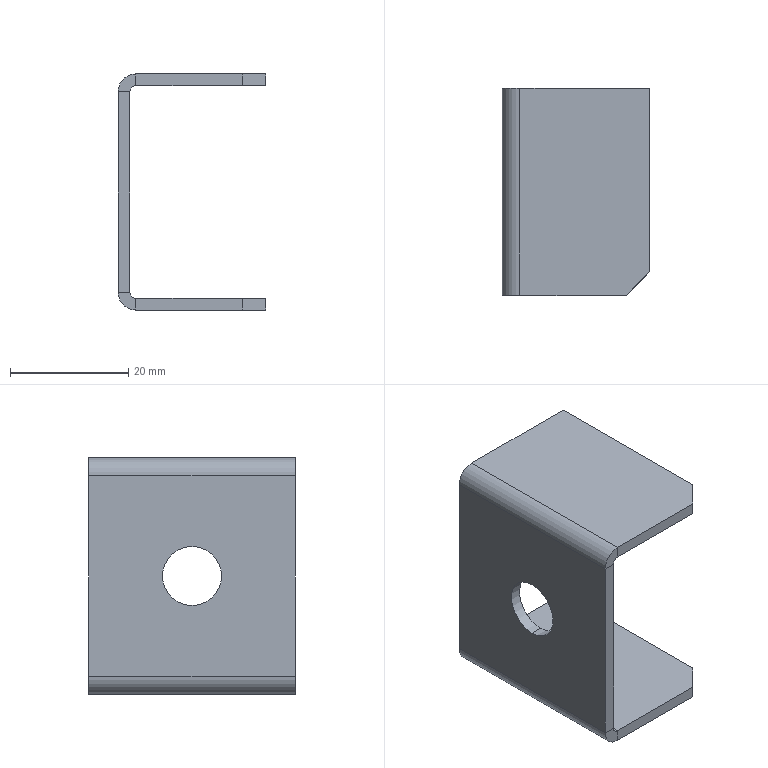Component | SolidWorks | GroundingDeviceAssembly-1_GroundingDevice-1 | 1 solid | 26 faces | box 25 x 35 x 40 mm | volume 5711 mm3 | plane 20 | cylinder 6 | commonest cylinder face diameters 10 x2 6 x2 2 x2
STEP:
#1=CARTESIAN_POINT('',(29.337,-7.169,9.724));
#2=VERTEX_POINT('',#1);
#3=CARTESIAN_POINT('',(29.337,-7.169,9.331));
#4=VERTEX_POINT('',#3);
#5=CARTESIAN_POINT('',(29.337,-7.169,9.528));
#6=DIRECTION('',(1.,0.,-0.));
#7=DIRECTION('',(0.,0.,-1.));
#8=AXIS2_PLACEMENT_3D('',#5,#6,#7);
#9=CIRCLE('',#8,0.1969);
#10=EDGE_CURVE('',#2,#4,#9,.T.);
#11=ORIENTED_EDGE('',*,*,#10,.T.);
#12=CARTESIAN_POINT('',(29.258,-7.169,9.331));
#13=VERTEX_POINT('',#12);
#14=CARTESIAN_POINT('',(29.376,-7.169,9.331));
#15=DIRECTION('',(-1.,-0.,0.));
#16=VECTOR('',#15,39.37);
#17=LINE('',#14,#16);
#18=EDGE_CURVE('',#4,#13,#17,.T.);
#19=ORIENTED_EDGE('',*,*,#18,.T.);
#20=CARTESIAN_POINT('',(29.258,-7.169,9.724));
#21=VERTEX_POINT('',#20);
#22=CARTESIAN_POINT('',(29.258,-7.169,9.528));
#23=DIRECTION('',(-1.,-0.,0.));
#24=DIRECTION('',(0.,0.,1.));
#25=AXIS2_PLACEMENT_3D('',#22,#23,#24);
#26=CIRCLE('',#25,0.1969);
#27=EDGE_CURVE('',#13,#21,#26,.T.);
#28=ORIENTED_EDGE('',*,*,#27,.T.);
#29=CARTESIAN_POINT('',(29.376,-7.169,9.724));
#30=DIRECTION('',(-1.,-0.,0.));
#31=VECTOR('',#30,39.37);
#32=LINE('',#29,#31);
#33=EDGE_CURVE('',#2,#21,#32,.T.);
#34=ORIENTED_EDGE('',*,*,#33,.F.);
#35=EDGE_LOOP('',(#11,#19,#28,#34));
#36=FACE_OUTER_BOUND('',#35,.T.);
#37=CARTESIAN_POINT('',(29.376,-7.169,9.528));
#38=DIRECTION('',(-1.,-0.,0.));
#39=DIRECTION('',(0.,0.,1.));
#40=AXIS2_PLACEMENT_3D('',#37,#38,#39);
#41=CYLINDRICAL_SURFACE('',#40,0.1969);
#42=ADVANCED_FACE('',(#36),#41,.F.);
#43=CARTESIAN_POINT('',(29.258,-7.169,9.528));
#44=DIRECTION('',(-1.,-0.,0.));
#45=DIRECTION('',(0.,0.,1.));
#46=AXIS2_PLACEMENT_3D('',#43,#44,#45);
#47=CIRCLE('',#46,0.1969);
#48=EDGE_CURVE('',#21,#13,#47,.T.);
#49=ORIENTED_EDGE('',*,*,#48,.F.);
#50=ORIENTED_EDGE('',*,*,#27,.F.);
#51=EDGE_LOOP('',(#49,#50));
#52=FACE_BOUND('',#51,.T.);
#53=CARTESIAN_POINT('',(29.258,-6.481,8.858));
#54=VERTEX_POINT('',#53);
#55=CARTESIAN_POINT('',(29.258,-7.858,8.858));
#56=VERTEX_POINT('',#55);
#57=CARTESIAN_POINT('',(29.258,-6.481,8.858));
#58=DIRECTION('',(0.,-1.,0.));
#59=VECTOR('',#58,39.37);
#60=LINE('',#57,#59);
#61=EDGE_CURVE('',#54,#56,#60,.T.);
#62=ORIENTED_EDGE('',*,*,#61,.T.);
#63=CARTESIAN_POINT('',(29.258,-7.858,10.197));
#64=VERTEX_POINT('',#63);
#65=CARTESIAN_POINT('',(29.258,-7.858,10.315));
#66=DIRECTION('',(-0.,-0.,-1.));
#67=VECTOR('',#66,39.37);
#68=LINE('',#65,#67);
#69=EDGE_CURVE('',#64,#56,#68,.T.);
#70=ORIENTED_EDGE('',*,*,#69,.F.);
#71=CARTESIAN_POINT('',(29.258,-6.481,10.197));
#72=VERTEX_POINT('',#71);
#73=CARTESIAN_POINT('',(29.258,-7.858,10.197));
#74=DIRECTION('',(-0.,1.,-0.));
#75=VECTOR('',#74,39.37);
#76=LINE('',#73,#75);
#77=EDGE_CURVE('',#64,#72,#76,.T.);
#78=ORIENTED_EDGE('',*,*,#77,.T.);
#79=CARTESIAN_POINT('',(29.258,-6.481,10.315));
#80=DIRECTION('',(0.,0.,1.));
#81=VECTOR('',#80,39.37);
#82=LINE('',#79,#81);
#83=EDGE_CURVE('',#54,#72,#82,.T.);
#84=ORIENTED_EDGE('',*,*,#83,.F.);
#85=EDGE_LOOP('',(#62,#70,#78,#84));
#86=FACE_OUTER_BOUND('',#85,.T.);
#87=CARTESIAN_POINT('',(29.258,-7.858,8.74));
#88=DIRECTION('',(1.,0.,-0.));
#89=DIRECTION('',(-0.,-0.,-1.));
#90=AXIS2_PLACEMENT_3D('',#87,#88,#89);
#91=PLANE('',#90);
#92=ADVANCED_FACE('',(#52,#86),#91,.F.);
#93=ORIENTED_EDGE('',*,*,#10,.F.);
#94=CARTESIAN_POINT('',(29.337,-7.169,9.528));
#95=DIRECTION('',(1.,0.,-0.));
#96=DIRECTION('',(0.,0.,-1.));
#97=AXIS2_PLACEMENT_3D('',#94,#95,#96);
#98=CIRCLE('',#97,0.1969);
#99=EDGE_CURVE('',#4,#2,#98,.T.);
#100=ORIENTED_EDGE('',*,*,#99,.F.);
#101=EDGE_LOOP('',(#93,#100));
#102=FACE_BOUND('',#101,.T.);
#103=CARTESIAN_POINT('',(29.337,-7.858,10.197));
#104=VERTEX_POINT('',#103);
#105=CARTESIAN_POINT('',(29.337,-7.858,8.858));
#106=VERTEX_POINT('',#105);
#107=CARTESIAN_POINT('',(29.337,-7.858,10.315));
#108=DIRECTION('',(-0.,-0.,-1.));
#109=VECTOR('',#108,39.37);
#110=LINE('',#107,#109);
#111=EDGE_CURVE('',#104,#106,#110,.T.);
#112=ORIENTED_EDGE('',*,*,#111,.T.);
#113=CARTESIAN_POINT('',(29.337,-6.481,8.858));
#114=VERTEX_POINT('',#113);
#115=CARTESIAN_POINT('',(29.337,-6.481,8.858));
#116=DIRECTION('',(0.,-1.,0.));
#117=VECTOR('',#116,39.37);
#118=LINE('',#115,#117);
#119=EDGE_CURVE('',#114,#106,#118,.T.);
#120=ORIENTED_EDGE('',*,*,#119,.F.);
#121=CARTESIAN_POINT('',(29.337,-6.481,10.197));
#122=VERTEX_POINT('',#121);
#123=CARTESIAN_POINT('',(29.337,-6.481,10.315));
#124=DIRECTION('',(0.,0.,1.));
#125=VECTOR('',#124,39.37);
#126=LINE('',#123,#125);
#127=EDGE_CURVE('',#114,#122,#126,.T.);
#128=ORIENTED_EDGE('',*,*,#127,.T.);
#129=CARTESIAN_POINT('',(29.337,-7.858,10.197));
#130=DIRECTION('',(-0.,1.,-0.));
#131=VECTOR('',#130,39.37);
#132=LINE('',#129,#131);
#133=EDGE_CURVE('',#104,#122,#132,.T.);
#134=ORIENTED_EDGE('',*,*,#133,.F.);
#135=EDGE_LOOP('',(#112,#120,#128,#134));
#136=FACE_OUTER_BOUND('',#135,.T.);
#137=CARTESIAN_POINT('',(29.337,-7.858,8.74));
#138=DIRECTION('',(1.,0.,-0.));
#139=DIRECTION('',(-0.,-0.,-1.));
#140=AXIS2_PLACEMENT_3D('',#137,#138,#139);
#141=PLANE('',#140);
#142=ADVANCED_FACE('',(#102,#136),#141,.T.);
#143=ORIENTED_EDGE('',*,*,#127,.F.);
#144=CARTESIAN_POINT('',(29.337,-6.481,8.858));
#145=DIRECTION('',(-1.,-0.,0.));
#146=VECTOR('',#145,39.37);
#147=LINE('',#144,#146);
#148=EDGE_CURVE('',#114,#54,#147,.T.);
#149=ORIENTED_EDGE('',*,*,#148,.T.);
#150=ORIENTED_EDGE('',*,*,#83,.T.);
#151=CARTESIAN_POINT('',(29.337,-6.481,10.197));
#152=DIRECTION('',(-1.,-0.,-0.));
#153=VECTOR('',#152,39.37);
#154=LINE('',#151,#153);
#155=EDGE_CURVE('',#122,#72,#154,.T.);
#156=ORIENTED_EDGE('',*,*,#155,.F.);
#157=EDGE_LOOP('',(#143,#149,#150,#156));
#158=FACE_OUTER_BOUND('',#157,.T.);
#159=CARTESIAN_POINT('',(29.258,-6.481,10.315));
#160=DIRECTION('',(-0.,1.,-0.));
#161=DIRECTION('',(1.,0.,-0.));
#162=AXIS2_PLACEMENT_3D('',#159,#160,#161);
#163=PLANE('',#162);
#164=ADVANCED_FACE('',(#158),#163,.T.);
#165=CARTESIAN_POINT('',(29.337,-7.858,8.858));
#166=DIRECTION('',(-1.,-0.,0.));
#167=VECTOR('',#166,39.37);
#168=LINE('',#165,#167);
#169=EDGE_CURVE('',#106,#56,#168,.T.);
#170=ORIENTED_EDGE('',*,*,#169,.F.);
#171=ORIENTED_EDGE('',*,*,#111,.F.);
#172=CARTESIAN_POINT('',(29.337,-7.858,10.197));
#173=DIRECTION('',(-1.,-0.,-0.));
#174=VECTOR('',#173,39.37);
#175=LINE('',#172,#174);
#176=EDGE_CURVE('',#104,#64,#175,.T.);
#177=ORIENTED_EDGE('',*,*,#176,.T.);
#178=ORIENTED_EDGE('',*,*,#69,.T.);
#179=EDGE_LOOP('',(#170,#171,#177,#178));
#180=FACE_OUTER_BOUND('',#179,.T.);
#181=CARTESIAN_POINT('',(29.258,-7.858,10.315));
#182=DIRECTION('',(0.,-1.,0.));
#183=DIRECTION('',(-1.,-0.,0.));
#184=AXIS2_PLACEMENT_3D('',#181,#182,#183);
#185=PLANE('',#184);
#186=ADVANCED_FACE('',(#180),#185,.T.);
#187=CARTESIAN_POINT('',(29.376,-6.481,10.236));
#188=VERTEX_POINT('',#187);
#189=CARTESIAN_POINT('',(29.376,-6.481,10.315));
#190=VERTEX_POINT('',#189);
#191=CARTESIAN_POINT('',(29.376,-6.481,10.315));
#192=DIRECTION('',(-0.,-0.,1.));
#193=VECTOR('',#192,39.37);
#194=LINE('',#191,#193);
#195=EDGE_CURVE('',#188,#190,#194,.T.);
#196=ORIENTED_EDGE('',*,*,#195,.F.);
#197=CARTESIAN_POINT('',(29.376,-6.481,10.197));
#198=DIRECTION('',(-0.,1.,-0.));
#199=DIRECTION('',(-1.,0.,0.));
#200=AXIS2_PLACEMENT_3D('',#197,#198,#199);
#201=CIRCLE('',#200,0.03937);
#202=EDGE_CURVE('',#122,#188,#201,.T.);
#203=ORIENTED_EDGE('',*,*,#202,.F.);
#204=ORIENTED_EDGE('',*,*,#155,.T.);
#205=CARTESIAN_POINT('',(29.376,-6.481,10.197));
#206=DIRECTION('',(-0.,1.,-0.));
#207=DIRECTION('',(-1.,0.,0.));
#208=AXIS2_PLACEMENT_3D('',#205,#206,#207);
#209=CIRCLE('',#208,0.1181);
#210=EDGE_CURVE('',#72,#190,#209,.T.);
#211=ORIENTED_EDGE('',*,*,#210,.T.);
#212=EDGE_LOOP('',(#196,#203,#204,#211));
#213=FACE_OUTER_BOUND('',#212,.T.);
#214=CARTESIAN_POINT('',(29.376,-6.481,10.197));
#215=DIRECTION('',(-0.,1.,-0.));
#216=DIRECTION('',(1.,0.,-0.));
#217=AXIS2_PLACEMENT_3D('',#214,#215,#216);
#218=PLANE('',#217);
#219=ADVANCED_FACE('',(#213),#218,.T.);
#220=CARTESIAN_POINT('',(29.376,-7.858,10.236));
#221=VERTEX_POINT('',#220);
#222=CARTESIAN_POINT('',(29.376,-7.858,10.197));
#223=DIRECTION('',(0.,-1.,0.));
#224=DIRECTION('',(-1.,0.,0.));
#225=AXIS2_PLACEMENT_3D('',#222,#223,#224);
#226=CIRCLE('',#225,0.03937);
#227=EDGE_CURVE('',#221,#104,#226,.T.);
#228=ORIENTED_EDGE('',*,*,#227,.F.);
#229=CARTESIAN_POINT('',(29.376,-7.858,10.315));
#230=VERTEX_POINT('',#229);
#231=CARTESIAN_POINT('',(29.376,-7.858,10.236));
#232=DIRECTION('',(-0.,-0.,1.));
#233=VECTOR('',#232,39.37);
#234=LINE('',#231,#233);
#235=EDGE_CURVE('',#221,#230,#234,.T.);
#236=ORIENTED_EDGE('',*,*,#235,.T.);
#237=CARTESIAN_POINT('',(29.376,-7.858,10.197));
#238=DIRECTION('',(0.,-1.,0.));
#239=DIRECTION('',(-1.,0.,0.));
#240=AXIS2_PLACEMENT_3D('',#237,#238,#239);
#241=CIRCLE('',#240,0.1181);
#242=EDGE_CURVE('',#230,#64,#241,.T.);
#243=ORIENTED_EDGE('',*,*,#242,.T.);
#244=ORIENTED_EDGE('',*,*,#176,.F.);
#245=EDGE_LOOP('',(#228,#236,#243,#244));
#246=FACE_OUTER_BOUND('',#245,.T.);
#247=CARTESIAN_POINT('',(29.376,-7.858,10.197));
#248=DIRECTION('',(-0.,1.,-0.));
#249=DIRECTION('',(1.,0.,-0.));
#250=AXIS2_PLACEMENT_3D('',#247,#248,#249);
#251=PLANE('',#250);
#252=ADVANCED_FACE('',(#246),#251,.F.);
#253=ORIENTED_EDGE('',*,*,#77,.F.);
#254=ORIENTED_EDGE('',*,*,#242,.F.);
#255=CARTESIAN_POINT('',(29.376,-6.481,10.315));
#256=DIRECTION('',(-0.,1.,-0.));
#257=VECTOR('',#256,39.37);
#258=LINE('',#255,#257);
#259=EDGE_CURVE('',#230,#190,#258,.T.);
#260=ORIENTED_EDGE('',*,*,#259,.T.);
#261=ORIENTED_EDGE('',*,*,#210,.F.);
#262=EDGE_LOOP('',(#253,#254,#260,#261));
#263=FACE_OUTER_BOUND('',#262,.T.);
#264=CARTESIAN_POINT('',(29.376,-7.858,10.197));
#265=DIRECTION('',(0.,-1.,0.));
#266=DIRECTION('',(0.,0.,1.));
#267=AXIS2_PLACEMENT_3D('',#264,#265,#266);
#268=CYLINDRICAL_SURFACE('',#267,0.1181);
#269=ADVANCED_FACE('',(#263),#268,.T.);
#270=ORIENTED_EDGE('',*,*,#133,.T.);
#271=ORIENTED_EDGE('',*,*,#202,.T.);
#272=CARTESIAN_POINT('',(29.376,-6.481,10.236));
#273=DIRECTION('',(0.,-1.,0.));
#274=VECTOR('',#273,39.37);
#275=LINE('',#272,#274);
#276=EDGE_CURVE('',#188,#221,#275,.T.);
#277=ORIENTED_EDGE('',*,*,#276,.T.);
#278=ORIENTED_EDGE('',*,*,#227,.T.);
#279=EDGE_LOOP('',(#270,#271,#277,#278));
#280=FACE_OUTER_BOUND('',#279,.T.);
#281=CARTESIAN_POINT('',(29.376,-7.858,10.197));
#282=DIRECTION('',(0.,-1.,0.));
#283=DIRECTION('',(0.,0.,1.));
#284=AXIS2_PLACEMENT_3D('',#281,#282,#283);
#285=CYLINDRICAL_SURFACE('',#284,0.03937);
#286=ADVANCED_FACE('',(#280),#285,.F.);
#287=ORIENTED_EDGE('',*,*,#195,.T.);
#288=CARTESIAN_POINT('',(30.242,-6.481,10.315));
#289=VERTEX_POINT('',#288);
#290=CARTESIAN_POINT('',(30.242,-6.481,10.315));
#291=DIRECTION('',(-1.,-0.,-0.));
#292=VECTOR('',#291,39.37);
#293=LINE('',#290,#292);
#294=EDGE_CURVE('',#289,#190,#293,.T.);
#295=ORIENTED_EDGE('',*,*,#294,.F.);
#296=CARTESIAN_POINT('',(30.242,-6.481,10.236));
#297=VERTEX_POINT('',#296);
#298=CARTESIAN_POINT('',(30.242,-6.481,10.315));
#299=DIRECTION('',(0.,0.,-1.));
#300=VECTOR('',#299,39.37);
#301=LINE('',#298,#300);
#302=EDGE_CURVE('',#289,#297,#301,.T.);
#303=ORIENTED_EDGE('',*,*,#302,.T.);
#304=CARTESIAN_POINT('',(29.337,-6.481,10.236));
#305=DIRECTION('',(-1.,-0.,-0.));
#306=VECTOR('',#305,39.37);
#307=LINE('',#304,#306);
#308=EDGE_CURVE('',#297,#188,#307,.T.);
#309=ORIENTED_EDGE('',*,*,#308,.T.);
#310=EDGE_LOOP('',(#287,#295,#303,#309));
#311=FACE_OUTER_BOUND('',#310,.T.);
#312=CARTESIAN_POINT('',(29.337,-6.481,10.315));
#313=DIRECTION('',(0.,-1.,-0.));
#314=DIRECTION('',(-0.,0.,-1.));
#315=AXIS2_PLACEMENT_3D('',#312,#313,#314);
#316=PLANE('',#315);
#317=ADVANCED_FACE('',(#311),#316,.F.);
#318=CARTESIAN_POINT('',(30.085,-7.858,10.236));
#319=VERTEX_POINT('',#318);
#320=CARTESIAN_POINT('',(30.242,-7.858,10.236));
#321=DIRECTION('',(1.,0.,0.));
#322=VECTOR('',#321,39.37);
#323=LINE('',#320,#322);
#324=EDGE_CURVE('',#221,#319,#323,.T.);
#325=ORIENTED_EDGE('',*,*,#324,.T.);
#326=CARTESIAN_POINT('',(30.085,-7.858,10.315));
#327=VERTEX_POINT('',#326);
#328=CARTESIAN_POINT('',(30.085,-7.858,10.315));
#329=DIRECTION('',(-0.,-0.,1.));
#330=VECTOR('',#329,39.37);
#331=LINE('',#328,#330);
#332=EDGE_CURVE('',#319,#327,#331,.T.);
#333=ORIENTED_EDGE('',*,*,#332,.T.);
#334=CARTESIAN_POINT('',(30.242,-7.858,10.315));
#335=DIRECTION('',(1.,0.,0.));
#336=VECTOR('',#335,39.37);
#337=LINE('',#334,#336);
#338=EDGE_CURVE('',#230,#327,#337,.T.);
#339=ORIENTED_EDGE('',*,*,#338,.F.);
#340=ORIENTED_EDGE('',*,*,#235,.F.);
#341=EDGE_LOOP('',(#325,#333,#339,#340));
#342=FACE_OUTER_BOUND('',#341,.T.);
#343=CARTESIAN_POINT('',(30.242,-7.858,10.315));
#344=DIRECTION('',(-0.,1.,0.));
#345=DIRECTION('',(0.,-0.,1.));
#346=AXIS2_PLACEMENT_3D('',#343,#344,#345);
#347=PLANE('',#346);
#348=ADVANCED_FACE('',(#342),#347,.F.);
#349=ORIENTED_EDGE('',*,*,#338,.T.);
#350=CARTESIAN_POINT('',(30.242,-7.701,10.315));
#351=VERTEX_POINT('',#350);
#352=CARTESIAN_POINT('',(30.242,-7.701,10.315));
#353=DIRECTION('',(0.7071,0.7071,0.));
#354=VECTOR('',#353,39.37);
#355=LINE('',#352,#354);
#356=EDGE_CURVE('',#327,#351,#355,.T.);
#357=ORIENTED_EDGE('',*,*,#356,.T.);
#358=CARTESIAN_POINT('',(30.242,-6.481,10.315));
#359=DIRECTION('',(-0.,1.,-0.));
#360=VECTOR('',#359,39.37);
#361=LINE('',#358,#360);
#362=EDGE_CURVE('',#351,#289,#361,.T.);
#363=ORIENTED_EDGE('',*,*,#362,.T.);
#364=ORIENTED_EDGE('',*,*,#294,.T.);
#365=ORIENTED_EDGE('',*,*,#259,.F.);
#366=EDGE_LOOP('',(#349,#357,#363,#364,#365));
#367=FACE_OUTER_BOUND('',#366,.T.);
#368=CARTESIAN_POINT('',(30.242,-6.481,10.315));
#369=DIRECTION('',(0.,0.,-1.));
#370=DIRECTION('',(-1.,-0.,-0.));
#371=AXIS2_PLACEMENT_3D('',#368,#369,#370);
#372=PLANE('',#371);
#373=ADVANCED_FACE('',(#367),#372,.F.);
#374=CARTESIAN_POINT('',(30.242,-7.701,10.236));
#375=VERTEX_POINT('',#374);
#376=CARTESIAN_POINT('',(30.242,-6.481,10.236));
#377=DIRECTION('',(-0.,1.,-0.));
#378=VECTOR('',#377,39.37);
#379=LINE('',#376,#378);
#380=EDGE_CURVE('',#375,#297,#379,.T.);
#381=ORIENTED_EDGE('',*,*,#380,.F.);
#382=CARTESIAN_POINT('',(30.852,-7.091,10.236));
#383=DIRECTION('',(-0.7071,-0.7071,-0.));
#384=VECTOR('',#383,39.37);
#385=LINE('',#382,#384);
#386=EDGE_CURVE('',#375,#319,#385,.T.);
#387=ORIENTED_EDGE('',*,*,#386,.T.);
#388=ORIENTED_EDGE('',*,*,#324,.F.);
#389=ORIENTED_EDGE('',*,*,#276,.F.);
#390=ORIENTED_EDGE('',*,*,#308,.F.);
#391=EDGE_LOOP('',(#381,#387,#388,#389,#390));
#392=FACE_OUTER_BOUND('',#391,.T.);
#393=CARTESIAN_POINT('',(30.242,-6.481,10.236));
#394=DIRECTION('',(0.,0.,-1.));
#395=DIRECTION('',(-1.,-0.,-0.));
#396=AXIS2_PLACEMENT_3D('',#393,#394,#395);
#397=PLANE('',#396);
#398=ADVANCED_FACE('',(#392),#397,.T.);
#399=ORIENTED_EDGE('',*,*,#362,.F.);
#400=CARTESIAN_POINT('',(30.242,-7.701,10.315));
#401=DIRECTION('',(0.,0.,-1.));
#402=VECTOR('',#401,39.37);
#403=LINE('',#400,#402);
#404=EDGE_CURVE('',#351,#375,#403,.T.);
#405=ORIENTED_EDGE('',*,*,#404,.T.);
#406=ORIENTED_EDGE('',*,*,#380,.T.);
#407=ORIENTED_EDGE('',*,*,#302,.F.);
#408=EDGE_LOOP('',(#399,#405,#406,#407));
#409=FACE_OUTER_BOUND('',#408,.T.);
#410=CARTESIAN_POINT('',(30.242,-6.481,10.315));
#411=DIRECTION('',(-1.,-0.,-0.));
#412=DIRECTION('',(-0.,0.,1.));
#413=AXIS2_PLACEMENT_3D('',#410,#411,#412);
#414=PLANE('',#413);
#415=ADVANCED_FACE('',(#409),#414,.F.);
#416=CARTESIAN_POINT('',(29.376,-7.858,8.819));
#417=VERTEX_POINT('',#416);
#418=CARTESIAN_POINT('',(29.376,-7.858,8.74));
#419=VERTEX_POINT('',#418);
#420=CARTESIAN_POINT('',(29.376,-7.858,8.74));
#421=DIRECTION('',(-0.,0.,-1.));
#422=VECTOR('',#421,39.37);
#423=LINE('',#420,#422);
#424=EDGE_CURVE('',#417,#419,#423,.T.);
#425=ORIENTED_EDGE('',*,*,#424,.F.);
#426=CARTESIAN_POINT('',(29.376,-7.858,8.858));
#427=DIRECTION('',(0.,-1.,0.));
#428=DIRECTION('',(1.,0.,0.));
#429=AXIS2_PLACEMENT_3D('',#426,#427,#428);
#430=CIRCLE('',#429,0.03937);
#431=EDGE_CURVE('',#106,#417,#430,.T.);
#432=ORIENTED_EDGE('',*,*,#431,.F.);
#433=ORIENTED_EDGE('',*,*,#169,.T.);
#434=CARTESIAN_POINT('',(29.376,-7.858,8.858));
#435=DIRECTION('',(0.,-1.,0.));
#436=DIRECTION('',(1.,0.,0.));
#437=AXIS2_PLACEMENT_3D('',#434,#435,#436);
#438=CIRCLE('',#437,0.1181);
#439=EDGE_CURVE('',#56,#419,#438,.T.);
#440=ORIENTED_EDGE('',*,*,#439,.T.);
#441=EDGE_LOOP('',(#425,#432,#433,#440));
#442=FACE_OUTER_BOUND('',#441,.T.);
#443=CARTESIAN_POINT('',(29.376,-7.858,8.858));
#444=DIRECTION('',(0.,-1.,0.));
#445=DIRECTION('',(-1.,-0.,0.));
#446=AXIS2_PLACEMENT_3D('',#443,#444,#445);
#447=PLANE('',#446);
#448=ADVANCED_FACE('',(#442),#447,.T.);
#449=CARTESIAN_POINT('',(29.376,-6.481,8.819));
#450=VERTEX_POINT('',#449);
#451=CARTESIAN_POINT('',(29.376,-6.481,8.858));
#452=DIRECTION('',(-0.,1.,-0.));
#453=DIRECTION('',(1.,0.,0.));
#454=AXIS2_PLACEMENT_3D('',#451,#452,#453);
#455=CIRCLE('',#454,0.03937);
#456=EDGE_CURVE('',#450,#114,#455,.T.);
#457=ORIENTED_EDGE('',*,*,#456,.F.);
#458=CARTESIAN_POINT('',(29.376,-6.481,8.74));
#459=VERTEX_POINT('',#458);
#460=CARTESIAN_POINT('',(29.376,-6.481,8.819));
#461=DIRECTION('',(-0.,0.,-1.));
#462=VECTOR('',#461,39.37);
#463=LINE('',#460,#462);
#464=EDGE_CURVE('',#450,#459,#463,.T.);
#465=ORIENTED_EDGE('',*,*,#464,.T.);
#466=CARTESIAN_POINT('',(29.376,-6.481,8.858));
#467=DIRECTION('',(-0.,1.,-0.));
#468=DIRECTION('',(1.,0.,0.));
#469=AXIS2_PLACEMENT_3D('',#466,#467,#468);
#470=CIRCLE('',#469,0.1181);
#471=EDGE_CURVE('',#459,#54,#470,.T.);
#472=ORIENTED_EDGE('',*,*,#471,.T.);
#473=ORIENTED_EDGE('',*,*,#148,.F.);
#474=EDGE_LOOP('',(#457,#465,#472,#473));
#475=FACE_OUTER_BOUND('',#474,.T.);
#476=CARTESIAN_POINT('',(29.376,-6.481,8.858));
#477=DIRECTION('',(0.,-1.,0.));
#478=DIRECTION('',(-1.,-0.,0.));
#479=AXIS2_PLACEMENT_3D('',#476,#477,#478);
#480=PLANE('',#479);
#481=ADVANCED_FACE('',(#475),#480,.F.);
#482=ORIENTED_EDGE('',*,*,#61,.F.);
#483=ORIENTED_EDGE('',*,*,#471,.F.);
#484=CARTESIAN_POINT('',(29.376,-7.858,8.74));
#485=DIRECTION('',(0.,-1.,0.));
#486=VECTOR('',#485,39.37);
#487=LINE('',#484,#486);
#488=EDGE_CURVE('',#459,#419,#487,.T.);
#489=ORIENTED_EDGE('',*,*,#488,.T.);
#490=ORIENTED_EDGE('',*,*,#439,.F.);
#491=EDGE_LOOP('',(#482,#483,#489,#490));
#492=FACE_OUTER_BOUND('',#491,.T.);
#493=CARTESIAN_POINT('',(29.376,-6.481,8.858));
#494=DIRECTION('',(-0.,1.,-0.));
#495=DIRECTION('',(0.,0.,-1.));
#496=AXIS2_PLACEMENT_3D('',#493,#494,#495);
#497=CYLINDRICAL_SURFACE('',#496,0.1181);
#498=ADVANCED_FACE('',(#492),#497,.T.);
#499=ORIENTED_EDGE('',*,*,#119,.T.);
#500=ORIENTED_EDGE('',*,*,#431,.T.);
#501=CARTESIAN_POINT('',(29.376,-7.858,8.819));
#502=DIRECTION('',(-0.,1.,-0.));
#503=VECTOR('',#502,39.37);
#504=LINE('',#501,#503);
#505=EDGE_CURVE('',#417,#450,#504,.T.);
#506=ORIENTED_EDGE('',*,*,#505,.T.);
#507=ORIENTED_EDGE('',*,*,#456,.T.);
#508=EDGE_LOOP('',(#499,#500,#506,#507));
#509=FACE_OUTER_BOUND('',#508,.T.);
#510=CARTESIAN_POINT('',(29.376,-6.481,8.858));
#511=DIRECTION('',(-0.,1.,-0.));
#512=DIRECTION('',(0.,0.,-1.));
#513=AXIS2_PLACEMENT_3D('',#510,#511,#512);
#514=CYLINDRICAL_SURFACE('',#513,0.03937);
#515=ADVANCED_FACE('',(#509),#514,.F.);
#516=CARTESIAN_POINT('',(30.085,-7.858,8.74));
#517=VERTEX_POINT('',#516);
#518=CARTESIAN_POINT('',(30.242,-7.858,8.74));
#519=DIRECTION('',(-1.,-0.,0.));
#520=VECTOR('',#519,39.37);
#521=LINE('',#518,#520);
#522=EDGE_CURVE('',#517,#419,#521,.T.);
#523=ORIENTED_EDGE('',*,*,#522,.F.);
#524=CARTESIAN_POINT('',(30.085,-7.858,8.819));
#525=VERTEX_POINT('',#524);
#526=CARTESIAN_POINT('',(30.085,-7.858,8.74));
#527=DIRECTION('',(0.,-0.,1.));
#528=VECTOR('',#527,39.37);
#529=LINE('',#526,#528);
#530=EDGE_CURVE('',#517,#525,#529,.T.);
#531=ORIENTED_EDGE('',*,*,#530,.T.);
#532=CARTESIAN_POINT('',(29.337,-7.858,8.819));
#533=DIRECTION('',(-1.,-0.,0.));
#534=VECTOR('',#533,39.37);
#535=LINE('',#532,#534);
#536=EDGE_CURVE('',#525,#417,#535,.T.);
#537=ORIENTED_EDGE('',*,*,#536,.T.);
#538=ORIENTED_EDGE('',*,*,#424,.T.);
#539=EDGE_LOOP('',(#523,#531,#537,#538));
#540=FACE_OUTER_BOUND('',#539,.T.);
#541=CARTESIAN_POINT('',(29.337,-7.858,8.74));
#542=DIRECTION('',(-0.,1.,0.));
#543=DIRECTION('',(0.,-0.,1.));
#544=AXIS2_PLACEMENT_3D('',#541,#542,#543);
#545=PLANE('',#544);
#546=ADVANCED_FACE('',(#540),#545,.F.);
#547=ORIENTED_EDGE('',*,*,#464,.F.);
#548=CARTESIAN_POINT('',(30.242,-6.481,8.819));
#549=VERTEX_POINT('',#548);
#550=CARTESIAN_POINT('',(30.242,-6.481,8.819));
#551=DIRECTION('',(1.,0.,-0.));
#552=VECTOR('',#551,39.37);
#553=LINE('',#550,#552);
#554=EDGE_CURVE('',#450,#549,#553,.T.);
#555=ORIENTED_EDGE('',*,*,#554,.T.);
#556=CARTESIAN_POINT('',(30.242,-6.481,8.74));
#557=VERTEX_POINT('',#556);
#558=CARTESIAN_POINT('',(30.242,-6.481,8.74));
#559=DIRECTION('',(0.,-0.,1.));
#560=VECTOR('',#559,39.37);
#561=LINE('',#558,#560);
#562=EDGE_CURVE('',#557,#549,#561,.T.);
#563=ORIENTED_EDGE('',*,*,#562,.F.);
#564=CARTESIAN_POINT('',(30.242,-6.481,8.74));
#565=DIRECTION('',(1.,0.,-0.));
#566=VECTOR('',#565,39.37);
#567=LINE('',#564,#566);
#568=EDGE_CURVE('',#459,#557,#567,.T.);
#569=ORIENTED_EDGE('',*,*,#568,.F.);
#570=EDGE_LOOP('',(#547,#555,#563,#569));
#571=FACE_OUTER_BOUND('',#570,.T.);
#572=CARTESIAN_POINT('',(30.242,-6.481,8.74));
#573=DIRECTION('',(0.,-1.,-0.));
#574=DIRECTION('',(-0.,0.,-1.));
#575=AXIS2_PLACEMENT_3D('',#572,#573,#574);
#576=PLANE('',#575);
#577=ADVANCED_FACE('',(#571),#576,.F.);
#578=CARTESIAN_POINT('',(30.242,-7.701,8.74));
#579=VERTEX_POINT('',#578);
#580=CARTESIAN_POINT('',(30.242,-7.858,8.74));
#581=DIRECTION('',(0.,-1.,0.));
#582=VECTOR('',#581,39.37);
#583=LINE('',#580,#582);
#584=EDGE_CURVE('',#557,#579,#583,.T.);
#585=ORIENTED_EDGE('',*,*,#584,.T.);
#586=CARTESIAN_POINT('',(30.085,-7.858,8.74));
#587=DIRECTION('',(-0.7071,-0.7071,0.));
#588=VECTOR('',#587,39.37);
#589=LINE('',#586,#588);
#590=EDGE_CURVE('',#579,#517,#589,.T.);
#591=ORIENTED_EDGE('',*,*,#590,.T.);
#592=ORIENTED_EDGE('',*,*,#522,.T.);
#593=ORIENTED_EDGE('',*,*,#488,.F.);
#594=ORIENTED_EDGE('',*,*,#568,.T.);
#595=EDGE_LOOP('',(#585,#591,#592,#593,#594));
#596=FACE_OUTER_BOUND('',#595,.T.);
#597=CARTESIAN_POINT('',(30.242,-7.858,8.74));
#598=DIRECTION('',(0.,-0.,1.));
#599=DIRECTION('',(1.,0.,-0.));
#600=AXIS2_PLACEMENT_3D('',#597,#598,#599);
#601=PLANE('',#600);
#602=ADVANCED_FACE('',(#596),#601,.F.);
#603=ORIENTED_EDGE('',*,*,#536,.F.);
#604=CARTESIAN_POINT('',(30.242,-7.701,8.819));
#605=VERTEX_POINT('',#604);
#606=CARTESIAN_POINT('',(30.163,-7.78,8.819));
#607=DIRECTION('',(0.7071,0.7071,-0.));
#608=VECTOR('',#607,39.37);
#609=LINE('',#606,#608);
#610=EDGE_CURVE('',#525,#605,#609,.T.);
#611=ORIENTED_EDGE('',*,*,#610,.T.);
#612=CARTESIAN_POINT('',(30.242,-7.858,8.819));
#613=DIRECTION('',(0.,-1.,0.));
#614=VECTOR('',#613,39.37);
#615=LINE('',#612,#614);
#616=EDGE_CURVE('',#549,#605,#615,.T.);
#617=ORIENTED_EDGE('',*,*,#616,.F.);
#618=ORIENTED_EDGE('',*,*,#554,.F.);
#619=ORIENTED_EDGE('',*,*,#505,.F.);
#620=EDGE_LOOP('',(#603,#611,#617,#618,#619));
#621=FACE_OUTER_BOUND('',#620,.T.);
#622=CARTESIAN_POINT('',(30.242,-7.858,8.819));
#623=DIRECTION('',(0.,-0.,1.));
#624=DIRECTION('',(1.,0.,-0.));
#625=AXIS2_PLACEMENT_3D('',#622,#623,#624);
#626=PLANE('',#625);
#627=ADVANCED_FACE('',(#621),#626,.T.);
#628=ORIENTED_EDGE('',*,*,#616,.T.);
#629=CARTESIAN_POINT('',(30.242,-7.701,8.74));
#630=DIRECTION('',(-0.,0.,-1.));
#631=VECTOR('',#630,39.37);
#632=LINE('',#629,#631);
#633=EDGE_CURVE('',#605,#579,#632,.T.);
#634=ORIENTED_EDGE('',*,*,#633,.T.);
#635=ORIENTED_EDGE('',*,*,#584,.F.);
#636=ORIENTED_EDGE('',*,*,#562,.T.);
#637=EDGE_LOOP('',(#628,#634,#635,#636));
#638=FACE_OUTER_BOUND('',#637,.T.);
#639=CARTESIAN_POINT('',(30.242,-7.858,8.74));
#640=DIRECTION('',(-1.,-0.,0.));
#641=DIRECTION('',(0.,0.,1.));
#642=AXIS2_PLACEMENT_3D('',#639,#640,#641);
#643=PLANE('',#642);
#644=ADVANCED_FACE('',(#638),#643,.F.);
#645=ORIENTED_EDGE('',*,*,#18,.F.);
#646=ORIENTED_EDGE('',*,*,#99,.T.);
#647=ORIENTED_EDGE('',*,*,#33,.T.);
#648=ORIENTED_EDGE('',*,*,#48,.T.);
#649=EDGE_LOOP('',(#645,#646,#647,#648));
#650=FACE_OUTER_BOUND('',#649,.T.);
#651=CARTESIAN_POINT('',(29.376,-7.169,9.528));
#652=DIRECTION('',(-1.,-0.,0.));
#653=DIRECTION('',(0.,0.,1.));
#654=AXIS2_PLACEMENT_3D('',#651,#652,#653);
#655=CYLINDRICAL_SURFACE('',#654,0.1969);
#656=ADVANCED_FACE('',(#650),#655,.F.);
#657=ORIENTED_EDGE('',*,*,#590,.F.);
#658=ORIENTED_EDGE('',*,*,#633,.F.);
#659=ORIENTED_EDGE('',*,*,#610,.F.);
#660=ORIENTED_EDGE('',*,*,#530,.F.);
#661=EDGE_LOOP('',(#657,#658,#659,#660));
#662=FACE_OUTER_BOUND('',#661,.T.);
#663=CARTESIAN_POINT('',(30.085,-7.858,8.74));
#664=DIRECTION('',(-0.7071,0.7071,0.));
#665=DIRECTION('',(0.,-0.,1.));
#666=AXIS2_PLACEMENT_3D('',#663,#664,#665);
#667=PLANE('',#666);
#668=ADVANCED_FACE('',(#662),#667,.F.);
#669=ORIENTED_EDGE('',*,*,#356,.F.);
#670=ORIENTED_EDGE('',*,*,#332,.F.);
#671=ORIENTED_EDGE('',*,*,#386,.F.);
#672=ORIENTED_EDGE('',*,*,#404,.F.);
#673=EDGE_LOOP('',(#669,#670,#671,#672));
#674=FACE_OUTER_BOUND('',#673,.T.);
#675=CARTESIAN_POINT('',(30.242,-7.701,10.315));
#676=DIRECTION('',(-0.7071,0.7071,-0.));
#677=DIRECTION('',(0.,0.,-1.));
#678=AXIS2_PLACEMENT_3D('',#675,#676,#677);
#679=PLANE('',#678);
#680=ADVANCED_FACE('',(#674),#679,.F.);
#681=CLOSED_SHELL('',(#42,#92,#142,#164,#186,#219,#252,#269,#286,#317,#348,#373,#398,#415,#448,#481,#498,#515,#546,#577,#602,#627,#644,#656,#668,#680));
#682=MANIFOLD_SOLID_BREP('',#681);
#683=CARTESIAN_POINT('',(0.,0.,0.));
#684=DIRECTION('',(0.,0.,1.));
#685=DIRECTION('',(1.,0.,0.));
#686=AXIS2_PLACEMENT_3D('',#683,#684,#685);
#687=(LENGTH_UNIT()NAMED_UNIT(*)SI_UNIT($,.METRE.));
#688=LENGTH_MEASURE_WITH_UNIT(LENGTH_MEASURE(0.0254),#687);
#689=DIMENSIONAL_EXPONENTS(1.,0.,0.,0.,0.,0.,0.);
#690=(CONVERSION_BASED_UNIT('',#688)LENGTH_UNIT()NAMED_UNIT(#689));
#691=UNCERTAINTY_MEASURE_WITH_UNIT(LENGTH_MEASURE(0.00001),#690,'','');
#692=(NAMED_UNIT(*)PLANE_ANGLE_UNIT()SI_UNIT($,.RADIAN.));
#693=(NAMED_UNIT(*)SI_UNIT($,.STERADIAN.)SOLID_ANGLE_UNIT());
#694=(GEOMETRIC_REPRESENTATION_CONTEXT(3)GLOBAL_UNCERTAINTY_ASSIGNED_CONTEXT((#691))GLOBAL_UNIT_ASSIGNED_CONTEXT((#690,#692,#693))REPRESENTATION_CONTEXT('',''));
#695=ADVANCED_BREP_SHAPE_REPRESENTATION('',(#682,#686),#694);
#696=COLOUR_RGB('',0.7922,0.8196,0.9333);
#697=FILL_AREA_STYLE_COLOUR('',#696);
#698=FILL_AREA_STYLE('',(#697));
#699=SURFACE_STYLE_FILL_AREA(#698);
#700=SURFACE_SIDE_STYLE('',(#699));
#701=SURFACE_STYLE_USAGE(.BOTH.,#700);
#702=PRESENTATION_STYLE_ASSIGNMENT((#701));
#703=STYLED_ITEM('',(#702),#682);
#704=PRESENTATION_LAYER_ASSIGNMENT('','',(#703));
#705=(LENGTH_UNIT()NAMED_UNIT(*)SI_UNIT($,.METRE.));
#706=LENGTH_MEASURE_WITH_UNIT(LENGTH_MEASURE(0.0254),#705);
#707=DIMENSIONAL_EXPONENTS(1.,0.,0.,0.,0.,0.,0.);
#708=(CONVERSION_BASED_UNIT('',#706)LENGTH_UNIT()NAMED_UNIT(#707));
#709=UNCERTAINTY_MEASURE_WITH_UNIT(LENGTH_MEASURE(0.00001),#708,'','');
#710=(NAMED_UNIT(*)PLANE_ANGLE_UNIT()SI_UNIT($,.RADIAN.));
#711=(NAMED_UNIT(*)SI_UNIT($,.STERADIAN.)SOLID_ANGLE_UNIT());
#712=(GEOMETRIC_REPRESENTATION_CONTEXT(3)GLOBAL_UNCERTAINTY_ASSIGNED_CONTEXT((#709))GLOBAL_UNIT_ASSIGNED_CONTEXT((#708,#710,#711))REPRESENTATION_CONTEXT('',''));
#713=MECHANICAL_DESIGN_GEOMETRIC_PRESENTATION_REPRESENTATION('',(#703),#712);